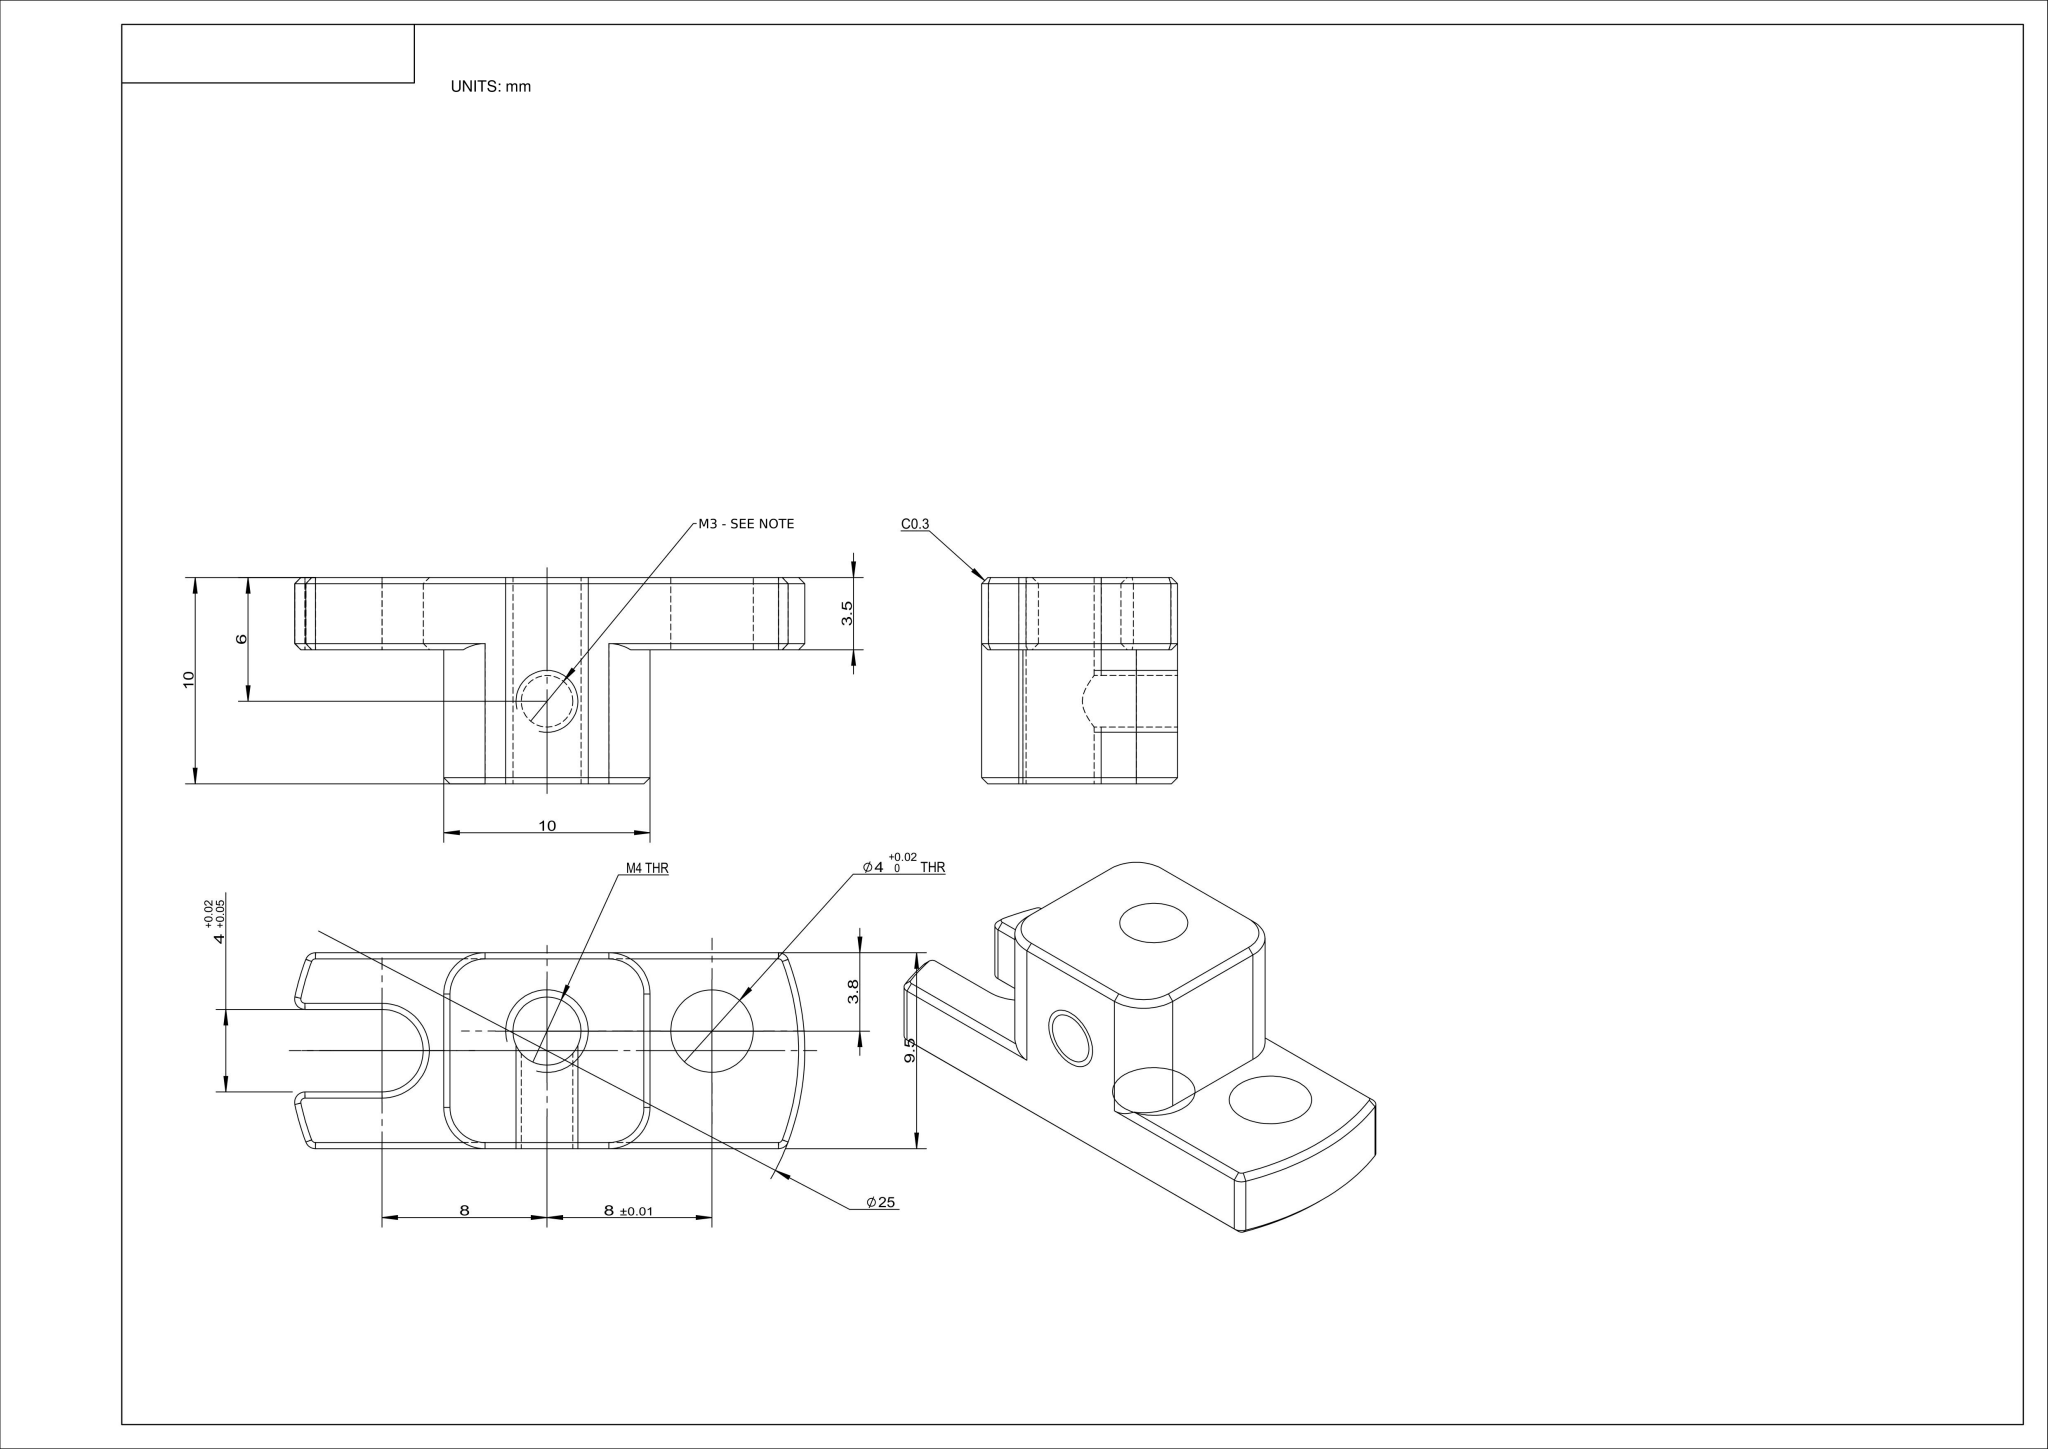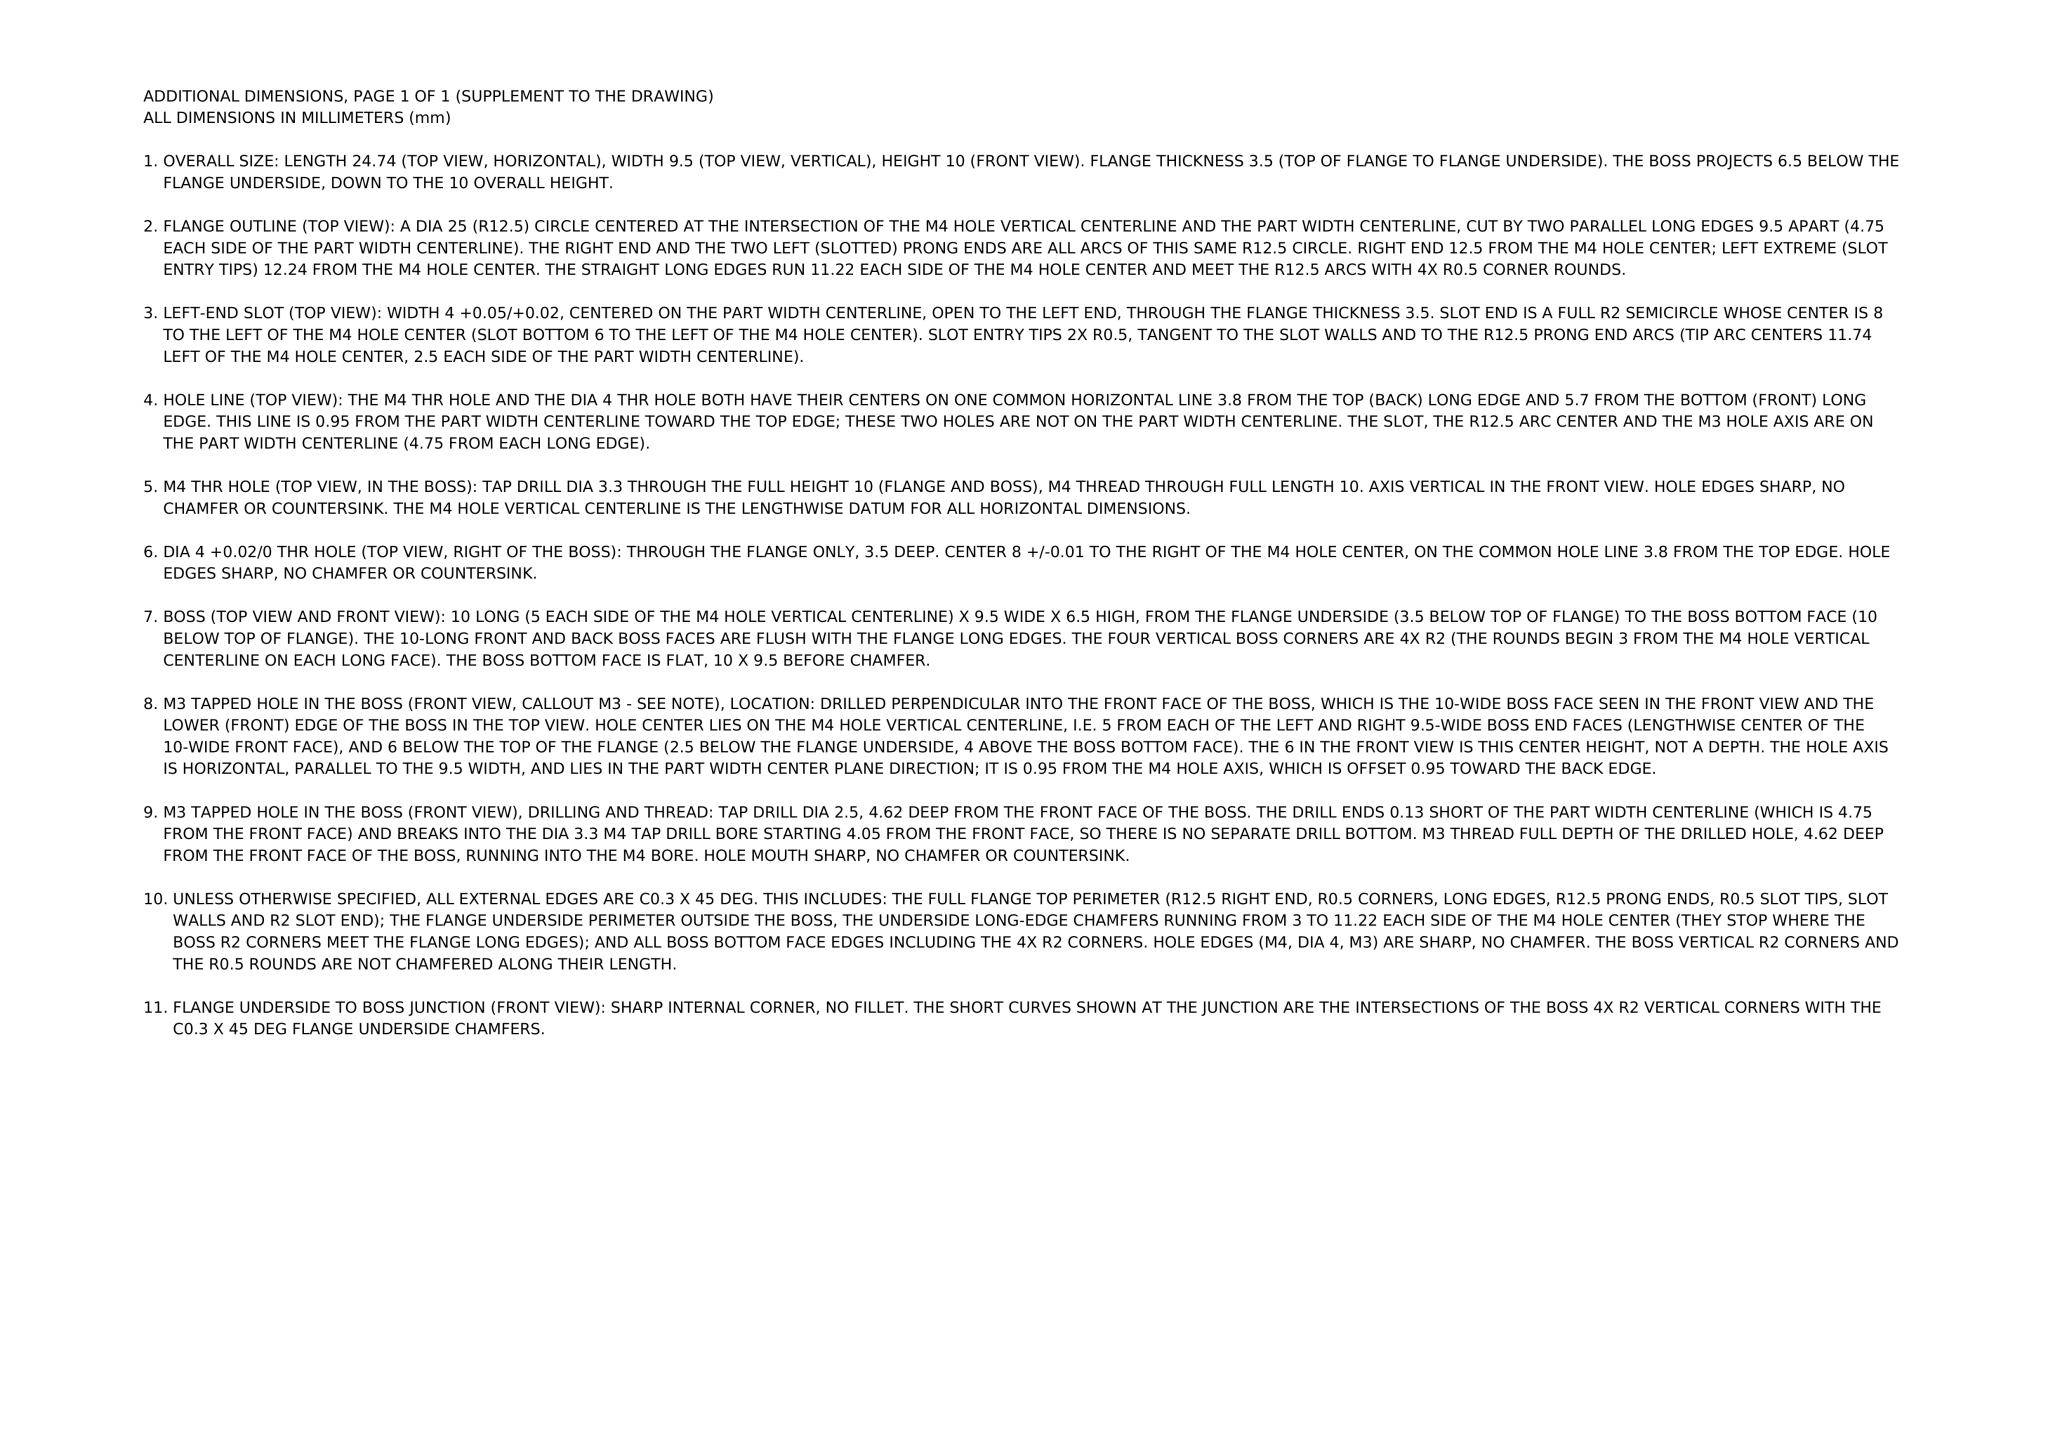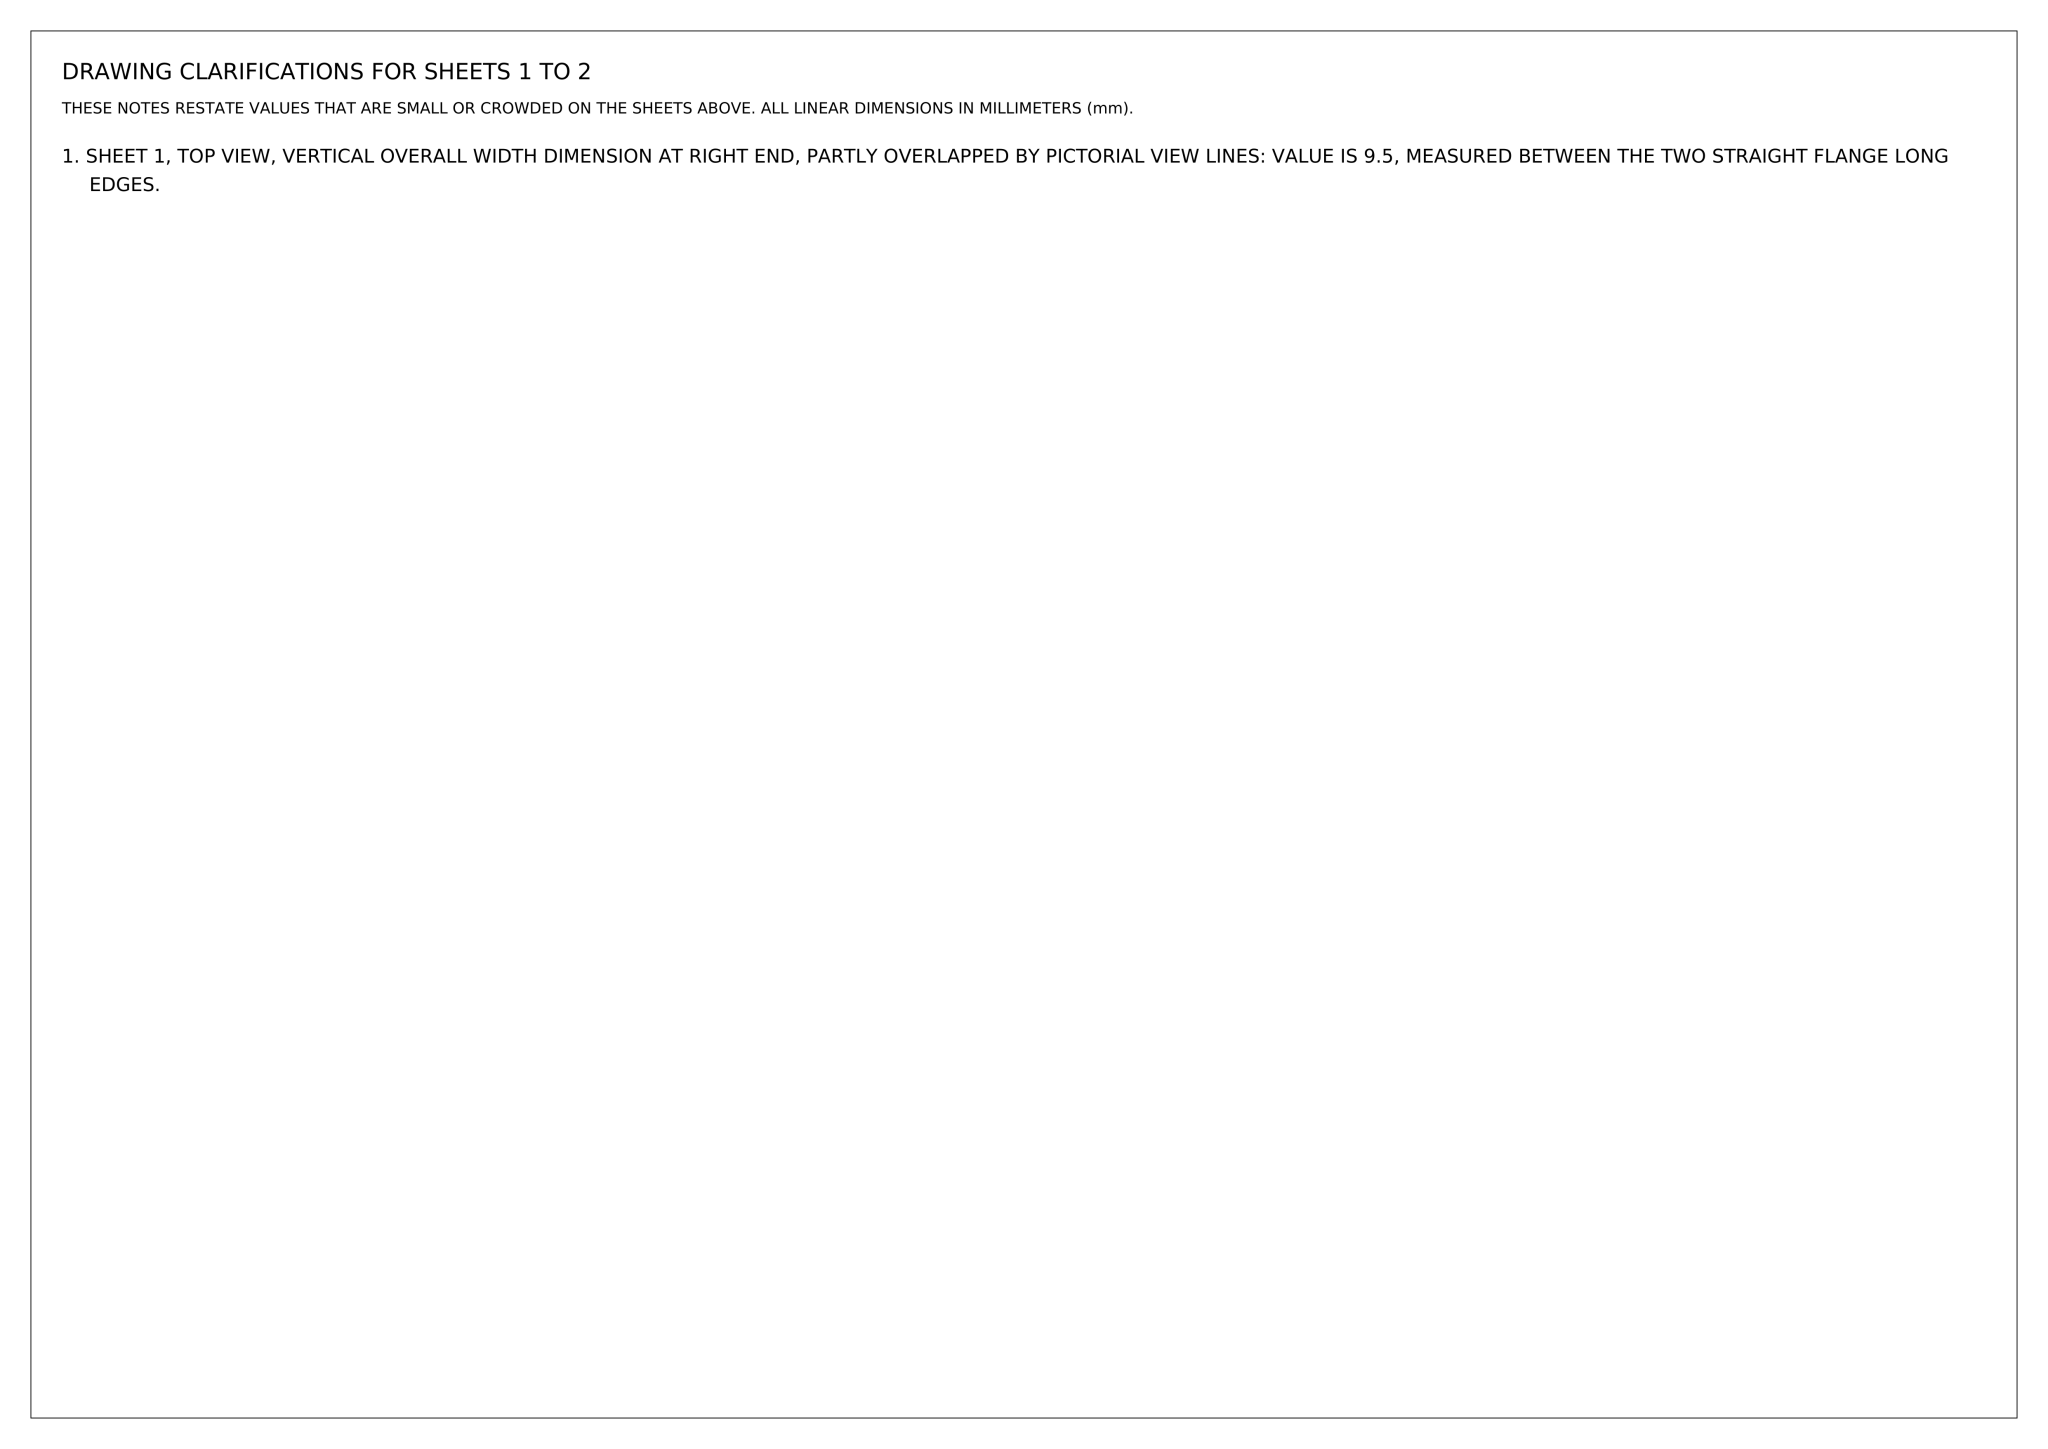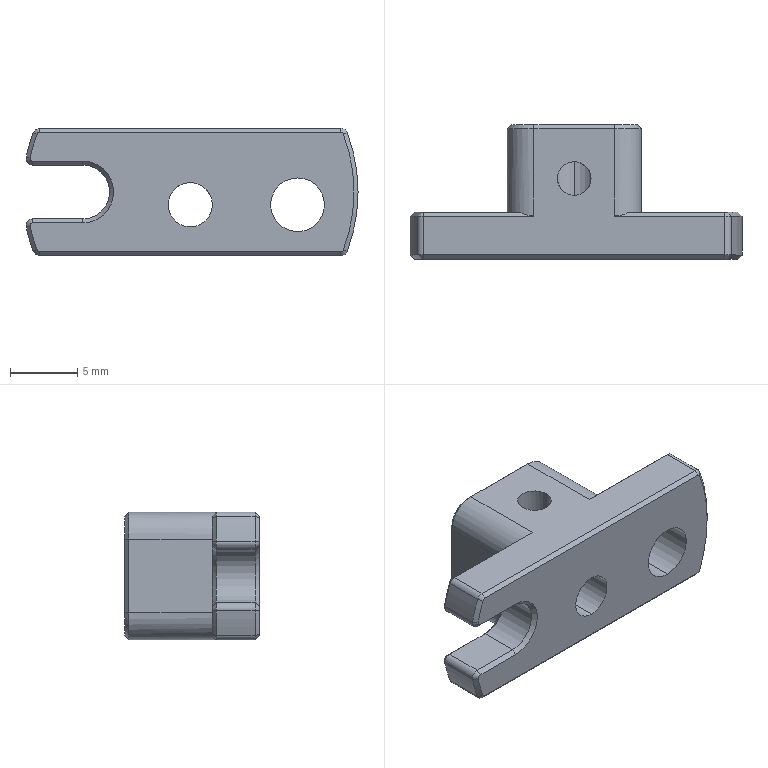Part | NX | mm | 1 solid | 68 faces | box 24.74 x 10 x 9.5 mm | volume 1163 mm3 | plane 24 | cone 24 | cylinder 20 | commonest cylinder face diameters 4 x7 1 x6 25 x3 2.5 x2 3.3 x2